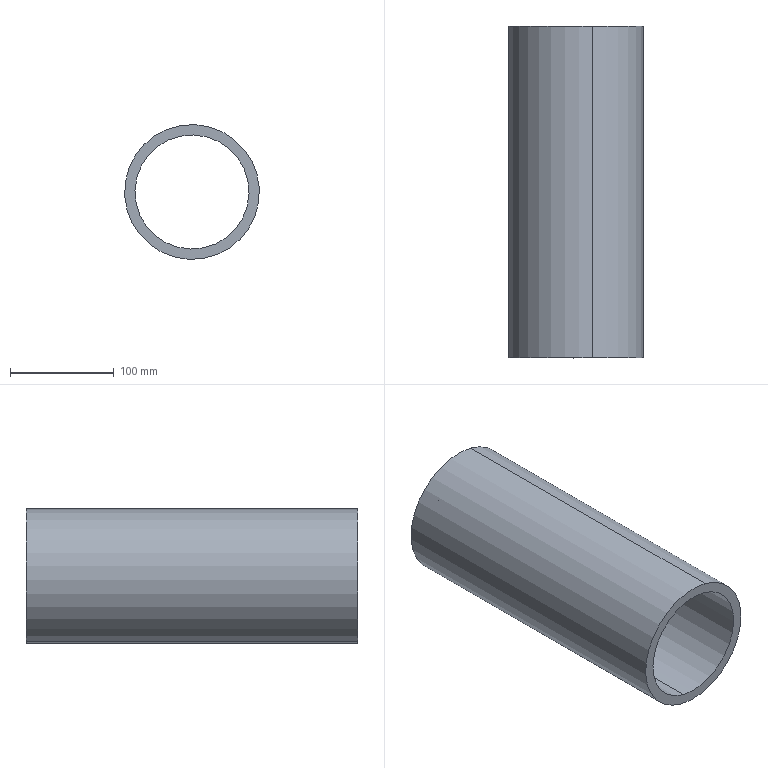Component | SolidWorks | FixedPost-1 | 1 solid | 22 faces | box 130 x 320 x 130 mm | volume 1202240 mm3 | cylinder 12 | cone 8 | plane 2 | commonest cylinder face diameters 8 x8 110 x2 130 x2
STEP:
#1=CARTESIAN_POINT('',(-5.204,20.011,23.757));
#2=VERTEX_POINT('',#1);
#3=CARTESIAN_POINT('',(-5.126,20.011,24.062));
#4=VERTEX_POINT('',#3);
#5=CARTESIAN_POINT('',(-5.165,20.011,23.91));
#6=DIRECTION('',(0.,1.,0.));
#7=DIRECTION('',(0.2479,0.,0.9688));
#8=AXIS2_PLACEMENT_3D('',#5,#6,#7);
#9=CIRCLE('',#8,0.1575);
#10=EDGE_CURVE('',#2,#4,#9,.T.);
#11=ORIENTED_EDGE('',*,*,#10,.F.);
#12=CARTESIAN_POINT('',(-5.204,20.788,23.757));
#13=VERTEX_POINT('',#12);
#14=CARTESIAN_POINT('',(-5.204,20.788,23.757));
#15=DIRECTION('',(0.,1.,0.));
#16=VECTOR('',#15,39.37);
#17=LINE('',#14,#16);
#18=EDGE_CURVE('',#2,#13,#17,.T.);
#19=ORIENTED_EDGE('',*,*,#18,.T.);
#20=CARTESIAN_POINT('',(-5.126,20.788,24.062));
#21=VERTEX_POINT('',#20);
#22=CARTESIAN_POINT('',(-5.165,20.788,23.91));
#23=DIRECTION('',(0.,1.,0.));
#24=DIRECTION('',(0.2479,0.,0.9688));
#25=AXIS2_PLACEMENT_3D('',#22,#23,#24);
#26=CIRCLE('',#25,0.1575);
#27=EDGE_CURVE('',#13,#21,#26,.T.);
#28=ORIENTED_EDGE('',*,*,#27,.T.);
#29=CARTESIAN_POINT('',(-5.126,20.788,24.062));
#30=DIRECTION('',(0.,1.,0.));
#31=VECTOR('',#30,39.37);
#32=LINE('',#29,#31);
#33=EDGE_CURVE('',#4,#21,#32,.T.);
#34=ORIENTED_EDGE('',*,*,#33,.F.);
#35=EDGE_LOOP('',(#11,#19,#28,#34));
#36=FACE_OUTER_BOUND('',#35,.T.);
#37=CARTESIAN_POINT('',(-5.165,20.788,23.91));
#38=DIRECTION('',(0.,1.,0.));
#39=DIRECTION('',(0.2479,0.,0.9688));
#40=AXIS2_PLACEMENT_3D('',#37,#38,#39);
#41=CYLINDRICAL_SURFACE('',#40,0.1575);
#42=ADVANCED_FACE('',(#36),#41,.F.);
#43=CARTESIAN_POINT('',(-5.165,19.916,23.91));
#44=VERTEX_POINT('',#43);
#45=CARTESIAN_POINT('',(-5.126,20.011,24.062));
#46=DIRECTION('',(0.2125,0.515,0.8304));
#47=VECTOR('',#46,39.37);
#48=LINE('',#45,#47);
#49=EDGE_CURVE('',#44,#4,#48,.T.);
#50=ORIENTED_EDGE('',*,*,#49,.F.);
#51=CARTESIAN_POINT('',(-5.204,20.011,23.757));
#52=DIRECTION('',(-0.2125,0.515,-0.8304));
#53=VECTOR('',#52,39.37);
#54=LINE('',#51,#53);
#55=EDGE_CURVE('',#44,#2,#54,.T.);
#56=ORIENTED_EDGE('',*,*,#55,.T.);
#57=ORIENTED_EDGE('',*,*,#10,.T.);
#58=EDGE_LOOP('',(#50,#56,#57));
#59=FACE_OUTER_BOUND('',#58,.T.);
#60=CARTESIAN_POINT('',(-5.165,20.011,23.91));
#61=DIRECTION('',(0.,1.,0.));
#62=DIRECTION('',(0.2479,0.,0.9688));
#63=AXIS2_PLACEMENT_3D('',#60,#61,#62);
#64=CONICAL_SURFACE('',#63,0.1575,1.03);
#65=ADVANCED_FACE('',(#59),#64,.F.);
#66=CARTESIAN_POINT('',(-1.865,20.011,23.874));
#67=VERTEX_POINT('',#66);
#68=CARTESIAN_POINT('',(-1.787,20.011,24.179));
#69=VERTEX_POINT('',#68);
#70=CARTESIAN_POINT('',(-1.826,20.011,24.026));
#71=DIRECTION('',(0.,1.,0.));
#72=DIRECTION('',(0.2479,0.,0.9688));
#73=AXIS2_PLACEMENT_3D('',#70,#71,#72);
#74=CIRCLE('',#73,0.1575);
#75=EDGE_CURVE('',#67,#69,#74,.T.);
#76=ORIENTED_EDGE('',*,*,#75,.F.);
#77=CARTESIAN_POINT('',(-1.865,20.788,23.874));
#78=VERTEX_POINT('',#77);
#79=CARTESIAN_POINT('',(-1.865,20.788,23.874));
#80=DIRECTION('',(0.,1.,0.));
#81=VECTOR('',#80,39.37);
#82=LINE('',#79,#81);
#83=EDGE_CURVE('',#67,#78,#82,.T.);
#84=ORIENTED_EDGE('',*,*,#83,.T.);
#85=CARTESIAN_POINT('',(-1.787,20.788,24.179));
#86=VERTEX_POINT('',#85);
#87=CARTESIAN_POINT('',(-1.826,20.788,24.026));
#88=DIRECTION('',(0.,1.,0.));
#89=DIRECTION('',(0.2479,0.,0.9688));
#90=AXIS2_PLACEMENT_3D('',#87,#88,#89);
#91=CIRCLE('',#90,0.1575);
#92=EDGE_CURVE('',#78,#86,#91,.T.);
#93=ORIENTED_EDGE('',*,*,#92,.T.);
#94=CARTESIAN_POINT('',(-1.787,20.788,24.179));
#95=DIRECTION('',(0.,1.,0.));
#96=VECTOR('',#95,39.37);
#97=LINE('',#94,#96);
#98=EDGE_CURVE('',#69,#86,#97,.T.);
#99=ORIENTED_EDGE('',*,*,#98,.F.);
#100=EDGE_LOOP('',(#76,#84,#93,#99));
#101=FACE_OUTER_BOUND('',#100,.T.);
#102=CARTESIAN_POINT('',(-1.826,20.788,24.026));
#103=DIRECTION('',(0.,1.,0.));
#104=DIRECTION('',(0.2479,0.,0.9688));
#105=AXIS2_PLACEMENT_3D('',#102,#103,#104);
#106=CYLINDRICAL_SURFACE('',#105,0.1575);
#107=ADVANCED_FACE('',(#101),#106,.F.);
#108=CARTESIAN_POINT('',(-1.826,19.916,24.026));
#109=VERTEX_POINT('',#108);
#110=CARTESIAN_POINT('',(-1.787,20.011,24.179));
#111=DIRECTION('',(0.2125,0.515,0.8304));
#112=VECTOR('',#111,39.37);
#113=LINE('',#110,#112);
#114=EDGE_CURVE('',#109,#69,#113,.T.);
#115=ORIENTED_EDGE('',*,*,#114,.F.);
#116=CARTESIAN_POINT('',(-1.865,20.011,23.874));
#117=DIRECTION('',(-0.2125,0.515,-0.8304));
#118=VECTOR('',#117,39.37);
#119=LINE('',#116,#118);
#120=EDGE_CURVE('',#109,#67,#119,.T.);
#121=ORIENTED_EDGE('',*,*,#120,.T.);
#122=ORIENTED_EDGE('',*,*,#75,.T.);
#123=EDGE_LOOP('',(#115,#121,#122));
#124=FACE_OUTER_BOUND('',#123,.T.);
#125=CARTESIAN_POINT('',(-1.826,20.011,24.026));
#126=DIRECTION('',(0.,1.,0.));
#127=DIRECTION('',(0.2479,0.,0.9688));
#128=AXIS2_PLACEMENT_3D('',#125,#126,#127);
#129=CONICAL_SURFACE('',#128,0.1575,1.03);
#130=ADVANCED_FACE('',(#124),#129,.F.);
#131=CARTESIAN_POINT('',(-1.749,20.011,20.535));
#132=VERTEX_POINT('',#131);
#133=CARTESIAN_POINT('',(-1.671,20.011,20.84));
#134=VERTEX_POINT('',#133);
#135=CARTESIAN_POINT('',(-1.71,20.011,20.688));
#136=DIRECTION('',(0.,1.,0.));
#137=DIRECTION('',(0.2479,0.,0.9688));
#138=AXIS2_PLACEMENT_3D('',#135,#136,#137);
#139=CIRCLE('',#138,0.1575);
#140=EDGE_CURVE('',#132,#134,#139,.T.);
#141=ORIENTED_EDGE('',*,*,#140,.F.);
#142=CARTESIAN_POINT('',(-1.749,20.788,20.535));
#143=VERTEX_POINT('',#142);
#144=CARTESIAN_POINT('',(-1.749,20.788,20.535));
#145=DIRECTION('',(0.,1.,0.));
#146=VECTOR('',#145,39.37);
#147=LINE('',#144,#146);
#148=EDGE_CURVE('',#132,#143,#147,.T.);
#149=ORIENTED_EDGE('',*,*,#148,.T.);
#150=CARTESIAN_POINT('',(-1.671,20.788,20.84));
#151=VERTEX_POINT('',#150);
#152=CARTESIAN_POINT('',(-1.71,20.788,20.688));
#153=DIRECTION('',(0.,1.,0.));
#154=DIRECTION('',(0.2479,0.,0.9688));
#155=AXIS2_PLACEMENT_3D('',#152,#153,#154);
#156=CIRCLE('',#155,0.1575);
#157=EDGE_CURVE('',#143,#151,#156,.T.);
#158=ORIENTED_EDGE('',*,*,#157,.T.);
#159=CARTESIAN_POINT('',(-1.671,20.788,20.84));
#160=DIRECTION('',(0.,1.,0.));
#161=VECTOR('',#160,39.37);
#162=LINE('',#159,#161);
#163=EDGE_CURVE('',#134,#151,#162,.T.);
#164=ORIENTED_EDGE('',*,*,#163,.F.);
#165=EDGE_LOOP('',(#141,#149,#158,#164));
#166=FACE_OUTER_BOUND('',#165,.T.);
#167=CARTESIAN_POINT('',(-1.71,20.788,20.688));
#168=DIRECTION('',(0.,1.,0.));
#169=DIRECTION('',(0.2479,0.,0.9688));
#170=AXIS2_PLACEMENT_3D('',#167,#168,#169);
#171=CYLINDRICAL_SURFACE('',#170,0.1575);
#172=ADVANCED_FACE('',(#166),#171,.F.);
#173=CARTESIAN_POINT('',(-1.71,19.916,20.688));
#174=VERTEX_POINT('',#173);
#175=CARTESIAN_POINT('',(-1.671,20.011,20.84));
#176=DIRECTION('',(0.2125,0.515,0.8304));
#177=VECTOR('',#176,39.37);
#178=LINE('',#175,#177);
#179=EDGE_CURVE('',#174,#134,#178,.T.);
#180=ORIENTED_EDGE('',*,*,#179,.F.);
#181=CARTESIAN_POINT('',(-1.749,20.011,20.535));
#182=DIRECTION('',(-0.2125,0.515,-0.8304));
#183=VECTOR('',#182,39.37);
#184=LINE('',#181,#183);
#185=EDGE_CURVE('',#174,#132,#184,.T.);
#186=ORIENTED_EDGE('',*,*,#185,.T.);
#187=ORIENTED_EDGE('',*,*,#140,.T.);
#188=EDGE_LOOP('',(#180,#186,#187));
#189=FACE_OUTER_BOUND('',#188,.T.);
#190=CARTESIAN_POINT('',(-1.71,20.011,20.688));
#191=DIRECTION('',(0.,1.,0.));
#192=DIRECTION('',(0.2479,0.,0.9688));
#193=AXIS2_PLACEMENT_3D('',#190,#191,#192);
#194=CONICAL_SURFACE('',#193,0.1575,1.03);
#195=ADVANCED_FACE('',(#189),#194,.F.);
#196=CARTESIAN_POINT('',(-5.087,20.011,20.419));
#197=VERTEX_POINT('',#196);
#198=CARTESIAN_POINT('',(-5.009,20.011,20.724));
#199=VERTEX_POINT('',#198);
#200=CARTESIAN_POINT('',(-5.048,20.011,20.571));
#201=DIRECTION('',(0.,1.,0.));
#202=DIRECTION('',(0.2479,0.,0.9688));
#203=AXIS2_PLACEMENT_3D('',#200,#201,#202);
#204=CIRCLE('',#203,0.1575);
#205=EDGE_CURVE('',#197,#199,#204,.T.);
#206=ORIENTED_EDGE('',*,*,#205,.F.);
#207=CARTESIAN_POINT('',(-5.087,20.788,20.419));
#208=VERTEX_POINT('',#207);
#209=CARTESIAN_POINT('',(-5.087,20.788,20.419));
#210=DIRECTION('',(0.,1.,0.));
#211=VECTOR('',#210,39.37);
#212=LINE('',#209,#211);
#213=EDGE_CURVE('',#197,#208,#212,.T.);
#214=ORIENTED_EDGE('',*,*,#213,.T.);
#215=CARTESIAN_POINT('',(-5.009,20.788,20.724));
#216=VERTEX_POINT('',#215);
#217=CARTESIAN_POINT('',(-5.048,20.788,20.571));
#218=DIRECTION('',(0.,1.,0.));
#219=DIRECTION('',(0.2479,0.,0.9688));
#220=AXIS2_PLACEMENT_3D('',#217,#218,#219);
#221=CIRCLE('',#220,0.1575);
#222=EDGE_CURVE('',#208,#216,#221,.T.);
#223=ORIENTED_EDGE('',*,*,#222,.T.);
#224=CARTESIAN_POINT('',(-5.009,20.788,20.724));
#225=DIRECTION('',(0.,1.,0.));
#226=VECTOR('',#225,39.37);
#227=LINE('',#224,#226);
#228=EDGE_CURVE('',#199,#216,#227,.T.);
#229=ORIENTED_EDGE('',*,*,#228,.F.);
#230=EDGE_LOOP('',(#206,#214,#223,#229));
#231=FACE_OUTER_BOUND('',#230,.T.);
#232=CARTESIAN_POINT('',(-5.048,20.788,20.571));
#233=DIRECTION('',(0.,1.,0.));
#234=DIRECTION('',(0.2479,0.,0.9688));
#235=AXIS2_PLACEMENT_3D('',#232,#233,#234);
#236=CYLINDRICAL_SURFACE('',#235,0.1575);
#237=ADVANCED_FACE('',(#231),#236,.F.);
#238=CARTESIAN_POINT('',(-5.048,19.916,20.571));
#239=VERTEX_POINT('',#238);
#240=CARTESIAN_POINT('',(-5.009,20.011,20.724));
#241=DIRECTION('',(0.2125,0.515,0.8304));
#242=VECTOR('',#241,39.37);
#243=LINE('',#240,#242);
#244=EDGE_CURVE('',#239,#199,#243,.T.);
#245=ORIENTED_EDGE('',*,*,#244,.F.);
#246=CARTESIAN_POINT('',(-5.087,20.011,20.419));
#247=DIRECTION('',(-0.2125,0.515,-0.8304));
#248=VECTOR('',#247,39.37);
#249=LINE('',#246,#248);
#250=EDGE_CURVE('',#239,#197,#249,.T.);
#251=ORIENTED_EDGE('',*,*,#250,.T.);
#252=ORIENTED_EDGE('',*,*,#205,.T.);
#253=EDGE_LOOP('',(#245,#251,#252));
#254=FACE_OUTER_BOUND('',#253,.T.);
#255=CARTESIAN_POINT('',(-5.048,20.011,20.571));
#256=DIRECTION('',(0.,1.,0.));
#257=DIRECTION('',(0.2479,0.,0.9688));
#258=AXIS2_PLACEMENT_3D('',#255,#256,#257);
#259=CONICAL_SURFACE('',#258,0.1575,1.03);
#260=ADVANCED_FACE('',(#254),#259,.F.);
#261=CARTESIAN_POINT('',(-3.974,20.788,20.201));
#262=VERTEX_POINT('',#261);
#263=CARTESIAN_POINT('',(-2.901,20.788,24.397));
#264=VERTEX_POINT('',#263);
#265=CARTESIAN_POINT('',(-3.437,20.788,22.299));
#266=DIRECTION('',(0.,1.,0.));
#267=DIRECTION('',(0.2479,0.,0.9688));
#268=AXIS2_PLACEMENT_3D('',#265,#266,#267);
#269=CIRCLE('',#268,2.165);
#270=EDGE_CURVE('',#262,#264,#269,.T.);
#271=ORIENTED_EDGE('',*,*,#270,.T.);
#272=CARTESIAN_POINT('',(-2.901,8.19,24.397));
#273=VERTEX_POINT('',#272);
#274=CARTESIAN_POINT('',(-2.901,20.788,24.397));
#275=DIRECTION('',(0.,-1.,0.));
#276=VECTOR('',#275,39.37);
#277=LINE('',#274,#276);
#278=EDGE_CURVE('',#264,#273,#277,.T.);
#279=ORIENTED_EDGE('',*,*,#278,.T.);
#280=CARTESIAN_POINT('',(-3.974,8.19,20.201));
#281=VERTEX_POINT('',#280);
#282=CARTESIAN_POINT('',(-3.437,8.19,22.299));
#283=DIRECTION('',(0.,1.,0.));
#284=DIRECTION('',(0.2479,0.,0.9688));
#285=AXIS2_PLACEMENT_3D('',#282,#283,#284);
#286=CIRCLE('',#285,2.165);
#287=EDGE_CURVE('',#281,#273,#286,.T.);
#288=ORIENTED_EDGE('',*,*,#287,.F.);
#289=CARTESIAN_POINT('',(-3.974,20.788,20.201));
#290=DIRECTION('',(0.,-1.,0.));
#291=VECTOR('',#290,39.37);
#292=LINE('',#289,#291);
#293=EDGE_CURVE('',#262,#281,#292,.T.);
#294=ORIENTED_EDGE('',*,*,#293,.F.);
#295=EDGE_LOOP('',(#271,#279,#288,#294));
#296=FACE_OUTER_BOUND('',#295,.T.);
#297=CARTESIAN_POINT('',(-3.437,20.788,22.299));
#298=DIRECTION('',(0.,-1.,0.));
#299=DIRECTION('',(-0.2479,0.,-0.9688));
#300=AXIS2_PLACEMENT_3D('',#297,#298,#299);
#301=CYLINDRICAL_SURFACE('',#300,2.165);
#302=ADVANCED_FACE('',(#296),#301,.F.);
#303=CARTESIAN_POINT('',(-2.803,20.788,24.778));
#304=VERTEX_POINT('',#303);
#305=CARTESIAN_POINT('',(-4.072,20.788,19.82));
#306=VERTEX_POINT('',#305);
#307=CARTESIAN_POINT('',(-3.437,20.788,22.299));
#308=DIRECTION('',(0.,1.,0.));
#309=DIRECTION('',(0.2479,0.,0.9688));
#310=AXIS2_PLACEMENT_3D('',#307,#308,#309);
#311=CIRCLE('',#310,2.559);
#312=EDGE_CURVE('',#304,#306,#311,.T.);
#313=ORIENTED_EDGE('',*,*,#312,.F.);
#314=CARTESIAN_POINT('',(-2.803,8.19,24.778));
#315=VERTEX_POINT('',#314);
#316=CARTESIAN_POINT('',(-2.803,20.788,24.778));
#317=DIRECTION('',(0.,-1.,0.));
#318=VECTOR('',#317,39.37);
#319=LINE('',#316,#318);
#320=EDGE_CURVE('',#304,#315,#319,.T.);
#321=ORIENTED_EDGE('',*,*,#320,.T.);
#322=CARTESIAN_POINT('',(-4.072,8.19,19.82));
#323=VERTEX_POINT('',#322);
#324=CARTESIAN_POINT('',(-3.437,8.19,22.299));
#325=DIRECTION('',(0.,1.,0.));
#326=DIRECTION('',(0.2479,0.,0.9688));
#327=AXIS2_PLACEMENT_3D('',#324,#325,#326);
#328=CIRCLE('',#327,2.559);
#329=EDGE_CURVE('',#315,#323,#328,.T.);
#330=ORIENTED_EDGE('',*,*,#329,.T.);
#331=CARTESIAN_POINT('',(-4.072,20.788,19.82));
#332=DIRECTION('',(0.,-1.,0.));
#333=VECTOR('',#332,39.37);
#334=LINE('',#331,#333);
#335=EDGE_CURVE('',#306,#323,#334,.T.);
#336=ORIENTED_EDGE('',*,*,#335,.F.);
#337=EDGE_LOOP('',(#313,#321,#330,#336));
#338=FACE_OUTER_BOUND('',#337,.T.);
#339=CARTESIAN_POINT('',(-3.437,20.788,22.299));
#340=DIRECTION('',(0.,-1.,0.));
#341=DIRECTION('',(-0.2479,0.,-0.9688));
#342=AXIS2_PLACEMENT_3D('',#339,#340,#341);
#343=CYLINDRICAL_SURFACE('',#342,2.559);
#344=ADVANCED_FACE('',(#338),#343,.T.);
#345=CARTESIAN_POINT('',(-5.165,20.788,23.91));
#346=DIRECTION('',(0.,1.,0.));
#347=DIRECTION('',(0.2479,0.,0.9688));
#348=AXIS2_PLACEMENT_3D('',#345,#346,#347);
#349=CIRCLE('',#348,0.1575);
#350=EDGE_CURVE('',#21,#13,#349,.T.);
#351=ORIENTED_EDGE('',*,*,#350,.F.);
#352=ORIENTED_EDGE('',*,*,#27,.F.);
#353=EDGE_LOOP('',(#351,#352));
#354=FACE_BOUND('',#353,.T.);
#355=CARTESIAN_POINT('',(-1.826,20.788,24.026));
#356=DIRECTION('',(0.,1.,0.));
#357=DIRECTION('',(0.2479,0.,0.9688));
#358=AXIS2_PLACEMENT_3D('',#355,#356,#357);
#359=CIRCLE('',#358,0.1575);
#360=EDGE_CURVE('',#86,#78,#359,.T.);
#361=ORIENTED_EDGE('',*,*,#360,.F.);
#362=ORIENTED_EDGE('',*,*,#92,.F.);
#363=EDGE_LOOP('',(#361,#362));
#364=FACE_BOUND('',#363,.T.);
#365=CARTESIAN_POINT('',(-1.71,20.788,20.688));
#366=DIRECTION('',(0.,1.,0.));
#367=DIRECTION('',(0.2479,0.,0.9688));
#368=AXIS2_PLACEMENT_3D('',#365,#366,#367);
#369=CIRCLE('',#368,0.1575);
#370=EDGE_CURVE('',#151,#143,#369,.T.);
#371=ORIENTED_EDGE('',*,*,#370,.F.);
#372=ORIENTED_EDGE('',*,*,#157,.F.);
#373=EDGE_LOOP('',(#371,#372));
#374=FACE_BOUND('',#373,.T.);
#375=CARTESIAN_POINT('',(-5.048,20.788,20.571));
#376=DIRECTION('',(0.,1.,0.));
#377=DIRECTION('',(0.2479,0.,0.9688));
#378=AXIS2_PLACEMENT_3D('',#375,#376,#377);
#379=CIRCLE('',#378,0.1575);
#380=EDGE_CURVE('',#216,#208,#379,.T.);
#381=ORIENTED_EDGE('',*,*,#380,.F.);
#382=ORIENTED_EDGE('',*,*,#222,.F.);
#383=EDGE_LOOP('',(#381,#382));
#384=FACE_BOUND('',#383,.T.);
#385=CARTESIAN_POINT('',(-3.437,20.788,22.299));
#386=DIRECTION('',(0.,1.,0.));
#387=DIRECTION('',(0.2479,0.,0.9688));
#388=AXIS2_PLACEMENT_3D('',#385,#386,#387);
#389=CIRCLE('',#388,2.559);
#390=EDGE_CURVE('',#306,#304,#389,.T.);
#391=ORIENTED_EDGE('',*,*,#390,.T.);
#392=ORIENTED_EDGE('',*,*,#312,.T.);
#393=EDGE_LOOP('',(#391,#392));
#394=FACE_OUTER_BOUND('',#393,.T.);
#395=ORIENTED_EDGE('',*,*,#270,.F.);
#396=CARTESIAN_POINT('',(-3.437,20.788,22.299));
#397=DIRECTION('',(0.,1.,0.));
#398=DIRECTION('',(0.2479,0.,0.9688));
#399=AXIS2_PLACEMENT_3D('',#396,#397,#398);
#400=CIRCLE('',#399,2.165);
#401=EDGE_CURVE('',#264,#262,#400,.T.);
#402=ORIENTED_EDGE('',*,*,#401,.F.);
#403=EDGE_LOOP('',(#395,#402));
#404=FACE_BOUND('',#403,.T.);
#405=CARTESIAN_POINT('',(-3.437,20.788,22.299));
#406=DIRECTION('',(0.,1.,0.));
#407=DIRECTION('',(0.2479,0.,0.9688));
#408=AXIS2_PLACEMENT_3D('',#405,#406,#407);
#409=PLANE('',#408);
#410=ADVANCED_FACE('',(#354,#364,#374,#384,#394,#404),#409,.T.);
#411=CARTESIAN_POINT('',(-3.437,8.19,22.299));
#412=DIRECTION('',(0.,1.,0.));
#413=DIRECTION('',(0.2479,0.,0.9688));
#414=AXIS2_PLACEMENT_3D('',#411,#412,#413);
#415=CIRCLE('',#414,2.559);
#416=EDGE_CURVE('',#323,#315,#415,.T.);
#417=ORIENTED_EDGE('',*,*,#416,.F.);
#418=ORIENTED_EDGE('',*,*,#329,.F.);
#419=EDGE_LOOP('',(#417,#418));
#420=FACE_OUTER_BOUND('',#419,.T.);
#421=ORIENTED_EDGE('',*,*,#287,.T.);
#422=CARTESIAN_POINT('',(-3.437,8.19,22.299));
#423=DIRECTION('',(0.,1.,0.));
#424=DIRECTION('',(0.2479,0.,0.9688));
#425=AXIS2_PLACEMENT_3D('',#422,#423,#424);
#426=CIRCLE('',#425,2.165);
#427=EDGE_CURVE('',#273,#281,#426,.T.);
#428=ORIENTED_EDGE('',*,*,#427,.T.);
#429=EDGE_LOOP('',(#421,#428));
#430=FACE_BOUND('',#429,.T.);
#431=CARTESIAN_POINT('',(-3.437,8.19,22.299));
#432=DIRECTION('',(0.,1.,0.));
#433=DIRECTION('',(0.2479,0.,0.9688));
#434=AXIS2_PLACEMENT_3D('',#431,#432,#433);
#435=PLANE('',#434);
#436=ADVANCED_FACE('',(#420,#430),#435,.F.);
#437=ORIENTED_EDGE('',*,*,#320,.F.);
#438=ORIENTED_EDGE('',*,*,#390,.F.);
#439=ORIENTED_EDGE('',*,*,#335,.T.);
#440=ORIENTED_EDGE('',*,*,#416,.T.);
#441=EDGE_LOOP('',(#437,#438,#439,#440));
#442=FACE_OUTER_BOUND('',#441,.T.);
#443=CARTESIAN_POINT('',(-3.437,20.788,22.299));
#444=DIRECTION('',(0.,-1.,0.));
#445=DIRECTION('',(-0.2479,0.,-0.9688));
#446=AXIS2_PLACEMENT_3D('',#443,#444,#445);
#447=CYLINDRICAL_SURFACE('',#446,2.559);
#448=ADVANCED_FACE('',(#442),#447,.T.);
#449=ORIENTED_EDGE('',*,*,#278,.F.);
#450=ORIENTED_EDGE('',*,*,#401,.T.);
#451=ORIENTED_EDGE('',*,*,#293,.T.);
#452=ORIENTED_EDGE('',*,*,#427,.F.);
#453=EDGE_LOOP('',(#449,#450,#451,#452));
#454=FACE_OUTER_BOUND('',#453,.T.);
#455=CARTESIAN_POINT('',(-3.437,20.788,22.299));
#456=DIRECTION('',(0.,-1.,0.));
#457=DIRECTION('',(-0.2479,0.,-0.9688));
#458=AXIS2_PLACEMENT_3D('',#455,#456,#457);
#459=CYLINDRICAL_SURFACE('',#458,2.165);
#460=ADVANCED_FACE('',(#454),#459,.F.);
#461=ORIENTED_EDGE('',*,*,#250,.F.);
#462=ORIENTED_EDGE('',*,*,#244,.T.);
#463=CARTESIAN_POINT('',(-5.048,20.011,20.571));
#464=DIRECTION('',(0.,1.,0.));
#465=DIRECTION('',(0.2479,0.,0.9688));
#466=AXIS2_PLACEMENT_3D('',#463,#464,#465);
#467=CIRCLE('',#466,0.1575);
#468=EDGE_CURVE('',#199,#197,#467,.T.);
#469=ORIENTED_EDGE('',*,*,#468,.T.);
#470=EDGE_LOOP('',(#461,#462,#469));
#471=FACE_OUTER_BOUND('',#470,.T.);
#472=CARTESIAN_POINT('',(-5.048,20.011,20.571));
#473=DIRECTION('',(0.,1.,0.));
#474=DIRECTION('',(0.2479,0.,0.9688));
#475=AXIS2_PLACEMENT_3D('',#472,#473,#474);
#476=CONICAL_SURFACE('',#475,0.1575,1.03);
#477=ADVANCED_FACE('',(#471),#476,.F.);
#478=ORIENTED_EDGE('',*,*,#213,.F.);
#479=ORIENTED_EDGE('',*,*,#468,.F.);
#480=ORIENTED_EDGE('',*,*,#228,.T.);
#481=ORIENTED_EDGE('',*,*,#380,.T.);
#482=EDGE_LOOP('',(#478,#479,#480,#481));
#483=FACE_OUTER_BOUND('',#482,.T.);
#484=CARTESIAN_POINT('',(-5.048,20.788,20.571));
#485=DIRECTION('',(0.,1.,0.));
#486=DIRECTION('',(0.2479,0.,0.9688));
#487=AXIS2_PLACEMENT_3D('',#484,#485,#486);
#488=CYLINDRICAL_SURFACE('',#487,0.1575);
#489=ADVANCED_FACE('',(#483),#488,.F.);
#490=ORIENTED_EDGE('',*,*,#185,.F.);
#491=ORIENTED_EDGE('',*,*,#179,.T.);
#492=CARTESIAN_POINT('',(-1.71,20.011,20.688));
#493=DIRECTION('',(0.,1.,0.));
#494=DIRECTION('',(0.2479,0.,0.9688));
#495=AXIS2_PLACEMENT_3D('',#492,#493,#494);
#496=CIRCLE('',#495,0.1575);
#497=EDGE_CURVE('',#134,#132,#496,.T.);
#498=ORIENTED_EDGE('',*,*,#497,.T.);
#499=EDGE_LOOP('',(#490,#491,#498));
#500=FACE_OUTER_BOUND('',#499,.T.);
#501=CARTESIAN_POINT('',(-1.71,20.011,20.688));
#502=DIRECTION('',(0.,1.,0.));
#503=DIRECTION('',(0.2479,0.,0.9688));
#504=AXIS2_PLACEMENT_3D('',#501,#502,#503);
#505=CONICAL_SURFACE('',#504,0.1575,1.03);
#506=ADVANCED_FACE('',(#500),#505,.F.);
#507=ORIENTED_EDGE('',*,*,#148,.F.);
#508=ORIENTED_EDGE('',*,*,#497,.F.);
#509=ORIENTED_EDGE('',*,*,#163,.T.);
#510=ORIENTED_EDGE('',*,*,#370,.T.);
#511=EDGE_LOOP('',(#507,#508,#509,#510));
#512=FACE_OUTER_BOUND('',#511,.T.);
#513=CARTESIAN_POINT('',(-1.71,20.788,20.688));
#514=DIRECTION('',(0.,1.,0.));
#515=DIRECTION('',(0.2479,0.,0.9688));
#516=AXIS2_PLACEMENT_3D('',#513,#514,#515);
#517=CYLINDRICAL_SURFACE('',#516,0.1575);
#518=ADVANCED_FACE('',(#512),#517,.F.);
#519=ORIENTED_EDGE('',*,*,#120,.F.);
#520=ORIENTED_EDGE('',*,*,#114,.T.);
#521=CARTESIAN_POINT('',(-1.826,20.011,24.026));
#522=DIRECTION('',(0.,1.,0.));
#523=DIRECTION('',(0.2479,0.,0.9688));
#524=AXIS2_PLACEMENT_3D('',#521,#522,#523);
#525=CIRCLE('',#524,0.1575);
#526=EDGE_CURVE('',#69,#67,#525,.T.);
#527=ORIENTED_EDGE('',*,*,#526,.T.);
#528=EDGE_LOOP('',(#519,#520,#527));
#529=FACE_OUTER_BOUND('',#528,.T.);
#530=CARTESIAN_POINT('',(-1.826,20.011,24.026));
#531=DIRECTION('',(0.,1.,0.));
#532=DIRECTION('',(0.2479,0.,0.9688));
#533=AXIS2_PLACEMENT_3D('',#530,#531,#532);
#534=CONICAL_SURFACE('',#533,0.1575,1.03);
#535=ADVANCED_FACE('',(#529),#534,.F.);
#536=ORIENTED_EDGE('',*,*,#83,.F.);
#537=ORIENTED_EDGE('',*,*,#526,.F.);
#538=ORIENTED_EDGE('',*,*,#98,.T.);
#539=ORIENTED_EDGE('',*,*,#360,.T.);
#540=EDGE_LOOP('',(#536,#537,#538,#539));
#541=FACE_OUTER_BOUND('',#540,.T.);
#542=CARTESIAN_POINT('',(-1.826,20.788,24.026));
#543=DIRECTION('',(0.,1.,0.));
#544=DIRECTION('',(0.2479,0.,0.9688));
#545=AXIS2_PLACEMENT_3D('',#542,#543,#544);
#546=CYLINDRICAL_SURFACE('',#545,0.1575);
#547=ADVANCED_FACE('',(#541),#546,.F.);
#548=ORIENTED_EDGE('',*,*,#55,.F.);
#549=ORIENTED_EDGE('',*,*,#49,.T.);
#550=CARTESIAN_POINT('',(-5.165,20.011,23.91));
#551=DIRECTION('',(0.,1.,0.));
#552=DIRECTION('',(0.2479,0.,0.9688));
#553=AXIS2_PLACEMENT_3D('',#550,#551,#552);
#554=CIRCLE('',#553,0.1575);
#555=EDGE_CURVE('',#4,#2,#554,.T.);
#556=ORIENTED_EDGE('',*,*,#555,.T.);
#557=EDGE_LOOP('',(#548,#549,#556));
#558=FACE_OUTER_BOUND('',#557,.T.);
#559=CARTESIAN_POINT('',(-5.165,20.011,23.91));
#560=DIRECTION('',(0.,1.,0.));
#561=DIRECTION('',(0.2479,0.,0.9688));
#562=AXIS2_PLACEMENT_3D('',#559,#560,#561);
#563=CONICAL_SURFACE('',#562,0.1575,1.03);
#564=ADVANCED_FACE('',(#558),#563,.F.);
#565=ORIENTED_EDGE('',*,*,#18,.F.);
#566=ORIENTED_EDGE('',*,*,#555,.F.);
#567=ORIENTED_EDGE('',*,*,#33,.T.);
#568=ORIENTED_EDGE('',*,*,#350,.T.);
#569=EDGE_LOOP('',(#565,#566,#567,#568));
#570=FACE_OUTER_BOUND('',#569,.T.);
#571=CARTESIAN_POINT('',(-5.165,20.788,23.91));
#572=DIRECTION('',(0.,1.,0.));
#573=DIRECTION('',(0.2479,0.,0.9688));
#574=AXIS2_PLACEMENT_3D('',#571,#572,#573);
#575=CYLINDRICAL_SURFACE('',#574,0.1575);
#576=ADVANCED_FACE('',(#570),#575,.F.);
#577=CLOSED_SHELL('',(#42,#65,#107,#130,#172,#195,#237,#260,#302,#344,#410,#436,#448,#460,#477,#489,#506,#518,#535,#547,#564,#576));
#578=MANIFOLD_SOLID_BREP('',#577);
#579=CARTESIAN_POINT('',(0.,0.,0.));
#580=DIRECTION('',(0.,0.,1.));
#581=DIRECTION('',(1.,0.,0.));
#582=AXIS2_PLACEMENT_3D('',#579,#580,#581);
#583=(LENGTH_UNIT()NAMED_UNIT(*)SI_UNIT($,.METRE.));
#584=LENGTH_MEASURE_WITH_UNIT(LENGTH_MEASURE(0.0254),#583);
#585=DIMENSIONAL_EXPONENTS(1.,0.,0.,0.,0.,0.,0.);
#586=(CONVERSION_BASED_UNIT('',#584)LENGTH_UNIT()NAMED_UNIT(#585));
#587=UNCERTAINTY_MEASURE_WITH_UNIT(LENGTH_MEASURE(0.00001),#586,'','');
#588=(NAMED_UNIT(*)PLANE_ANGLE_UNIT()SI_UNIT($,.RADIAN.));
#589=(NAMED_UNIT(*)SI_UNIT($,.STERADIAN.)SOLID_ANGLE_UNIT());
#590=(GEOMETRIC_REPRESENTATION_CONTEXT(3)GLOBAL_UNCERTAINTY_ASSIGNED_CONTEXT((#587))GLOBAL_UNIT_ASSIGNED_CONTEXT((#586,#588,#589))REPRESENTATION_CONTEXT('',''));
#591=ADVANCED_BREP_SHAPE_REPRESENTATION('',(#578,#582),#590);
#592=COLOUR_RGB('',0.7922,0.8196,0.9333);
#593=FILL_AREA_STYLE_COLOUR('',#592);
#594=FILL_AREA_STYLE('',(#593));
#595=SURFACE_STYLE_FILL_AREA(#594);
#596=SURFACE_SIDE_STYLE('',(#595));
#597=SURFACE_STYLE_USAGE(.BOTH.,#596);
#598=PRESENTATION_STYLE_ASSIGNMENT((#597));
#599=STYLED_ITEM('',(#598),#578);
#600=PRESENTATION_LAYER_ASSIGNMENT('','',(#599));
#601=(LENGTH_UNIT()NAMED_UNIT(*)SI_UNIT($,.METRE.));
#602=LENGTH_MEASURE_WITH_UNIT(LENGTH_MEASURE(0.0254),#601);
#603=DIMENSIONAL_EXPONENTS(1.,0.,0.,0.,0.,0.,0.);
#604=(CONVERSION_BASED_UNIT('',#602)LENGTH_UNIT()NAMED_UNIT(#603));
#605=UNCERTAINTY_MEASURE_WITH_UNIT(LENGTH_MEASURE(0.00001),#604,'','');
#606=(NAMED_UNIT(*)PLANE_ANGLE_UNIT()SI_UNIT($,.RADIAN.));
#607=(NAMED_UNIT(*)SI_UNIT($,.STERADIAN.)SOLID_ANGLE_UNIT());
#608=(GEOMETRIC_REPRESENTATION_CONTEXT(3)GLOBAL_UNCERTAINTY_ASSIGNED_CONTEXT((#605))GLOBAL_UNIT_ASSIGNED_CONTEXT((#604,#606,#607))REPRESENTATION_CONTEXT('',''));
#609=MECHANICAL_DESIGN_GEOMETRIC_PRESENTATION_REPRESENTATION('',(#599),#608);